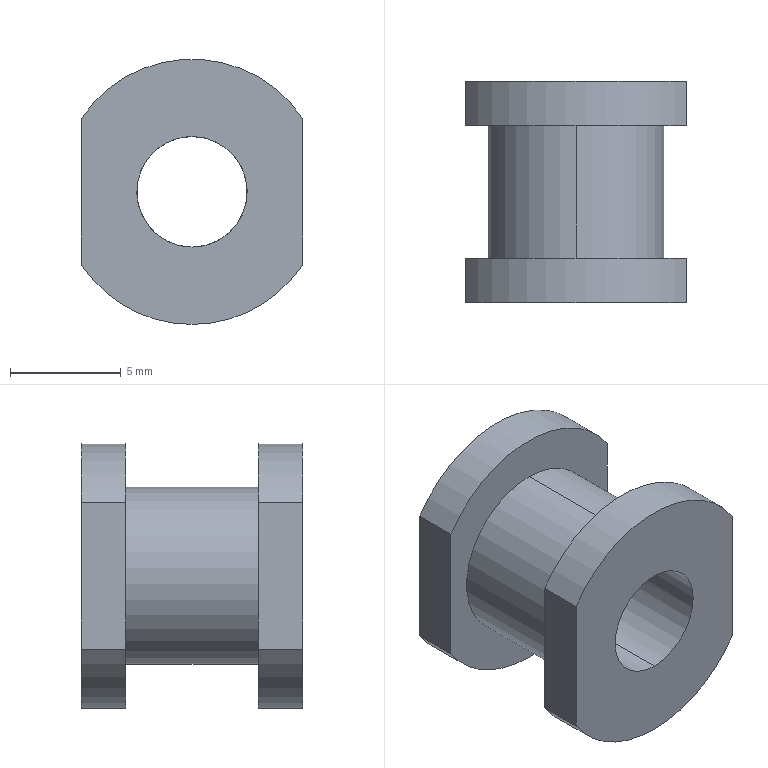Component | SolidWorks | F01AE00021-D54313-1 | 1 solid | 18 faces | box 10 x 10 x 12 mm | volume 522 mm3 | cylinder 10 | plane 8 | commonest cylinder face diameters 12 x6 5 x2 8 x2
build123d program:
from build123d import *

# Parameters (mm, degrees)
CUT_EXTRUDE1_DEPTH              = 10
M5_TAPPED_HOLE1_D               = 4.2
M5_TAPPED_HOLE1_DEPTH           = 12.4
M5_TAPPED_HOLE1_TIP             = 1.262
M5_THREADMAJORRELIEF_DEPTH      = 13.689
M5_THREADMAJORRELIEF_DEPTH_BACK = 13.689
M5_THREADMAJORRELIEF_SKETCH_R   = 2.5


with BuildPart() as part:
    # Sketch1 → Revolve1 (revolve)
    with BuildSketch(Plane.XY, mode=Mode.PRIVATE) as revolve1_sk:
        Polygon((2, 10), (2, 0), (6, 0), (6, 2), (4, 2), (4, 8), (6, 8), (6, 10), align=None)
    revolve(revolve1_sk.sketch.rotate(Axis((0, 0, 0), (0, 1, 0)), 90), axis=Axis((0, 0, 0), (0, 1, 0)))

    # Sketch2 → Cut-Extrude1 (cut)
    with BuildSketch(Plane(origin=(0, 10, 0), x_dir=(1, 0, 0), z_dir=(0, 1, 0))):
        with BuildLine():
            Line((-5, 3.317), (-5, -3.317))
            ThreePointArc((-5, -3.317), (-6, 0), (-5, 3.317))
        make_face()
        with BuildLine():
            Line((5, 3.317), (5, -3.317))
            ThreePointArc((5, -3.317), (6, 0), (5, 3.317))
        make_face()
    extrude(amount=-CUT_EXTRUDE1_DEPTH, mode=Mode.SUBTRACT)

    # M5 Tapped Hole1
    with Locations(Plane(origin=(0, 10, 0), x_dir=(1, 0, 0), z_dir=(0, 1, 0))):
        with Locations((0, 0)):
            Hole(M5_TAPPED_HOLE1_D / 2, depth=M5_TAPPED_HOLE1_DEPTH)
            with Locations((0, 0, -(M5_TAPPED_HOLE1_DEPTH + M5_TAPPED_HOLE1_TIP / 2))):  # 118° drill point
                Cone(0, M5_TAPPED_HOLE1_D / 2, M5_TAPPED_HOLE1_TIP, mode=Mode.SUBTRACT)

    # M5_ThreadMajorRelief_Sketch → M5_ThreadMajorRelief (cut, two sides: drawn at the far end of the back side and taken through both)
    with BuildSketch(Plane(origin=(0, 0, 0), x_dir=(1, 0, 0), z_dir=(0, 1, 0)).offset(-M5_THREADMAJORRELIEF_DEPTH_BACK)):
        with Locations(Location((0, 0, 0), (0, 0, 270))):
            Circle(M5_THREADMAJORRELIEF_SKETCH_R)
    extrude(amount=M5_THREADMAJORRELIEF_DEPTH + M5_THREADMAJORRELIEF_DEPTH_BACK, mode=Mode.SUBTRACT)


solid = part.part

# Placed as in the assembly
solid = solid.moved(Location((272.334, 153.205, 237.764), (0, 0, 0)))
STEP:
#1=COLOUR_RGB('',0.7922,0.8196,0.9333);
#2=FILL_AREA_STYLE_COLOUR('',#1);
#3=FILL_AREA_STYLE('',(#2));
#4=SURFACE_STYLE_FILL_AREA(#3);
#5=SURFACE_SIDE_STYLE('',(#4));
#6=SURFACE_STYLE_USAGE(.BOTH.,#5);
#7=PRESENTATION_STYLE_ASSIGNMENT((#6));
#8=CARTESIAN_POINT('',(10.722,6.032,9.262));
#9=VERTEX_POINT('',#8);
#10=CARTESIAN_POINT('',(10.722,6.032,9.459));
#11=VERTEX_POINT('',#10);
#12=CARTESIAN_POINT('',(10.722,6.032,9.262));
#13=CARTESIAN_POINT('',(10.709,6.032,9.262));
#14=CARTESIAN_POINT('',(10.696,6.032,9.265));
#15=CARTESIAN_POINT('',(10.672,6.032,9.275));
#16=CARTESIAN_POINT('',(10.661,6.032,9.282));
#17=CARTESIAN_POINT('',(10.643,6.032,9.3));
#18=CARTESIAN_POINT('',(10.636,6.032,9.311));
#19=CARTESIAN_POINT('',(10.626,6.032,9.335));
#20=CARTESIAN_POINT('',(10.623,6.032,9.348));
#21=CARTESIAN_POINT('',(10.623,6.032,9.374));
#22=CARTESIAN_POINT('',(10.626,6.032,9.386));
#23=CARTESIAN_POINT('',(10.636,6.032,9.411));
#24=CARTESIAN_POINT('',(10.643,6.032,9.421));
#25=CARTESIAN_POINT('',(10.661,6.032,9.44));
#26=CARTESIAN_POINT('',(10.672,6.032,9.447));
#27=CARTESIAN_POINT('',(10.696,6.032,9.457));
#28=CARTESIAN_POINT('',(10.709,6.032,9.459));
#29=CARTESIAN_POINT('',(10.722,6.032,9.459));
#30=B_SPLINE_CURVE_WITH_KNOTS('',3,(#12,#13,#14,#15,#16,#17,#18,#19,#20,#21,#22,#23,#24,#25,#26,#27,#28,#29),.UNSPECIFIED.,.F.,.F.,(4,2,2,2,2,2,2,2,4),(0.5,0.5625,0.625,0.6875,0.75,0.8125,0.875,0.9375,1.),.UNSPECIFIED.);
#31=EDGE_CURVE('',#9,#11,#30,.T.);
#32=ORIENTED_EDGE('',*,*,#31,.F.);
#33=CARTESIAN_POINT('',(10.722,6.425,9.262));
#34=VERTEX_POINT('',#33);
#35=CARTESIAN_POINT('',(10.722,6.032,9.262));
#36=DIRECTION('',(0.,1.,0.));
#37=VECTOR('',#36,39.37);
#38=LINE('',#35,#37);
#39=EDGE_CURVE('',#9,#34,#38,.T.);
#40=ORIENTED_EDGE('',*,*,#39,.T.);
#41=CARTESIAN_POINT('',(10.722,6.425,9.459));
#42=VERTEX_POINT('',#41);
#43=CARTESIAN_POINT('',(10.722,6.425,9.361));
#44=DIRECTION('',(0.,1.,0.));
#45=DIRECTION('',(0.,0.,1.));
#46=AXIS2_PLACEMENT_3D('',#43,#44,#45);
#47=CIRCLE('',#46,0.09843);
#48=EDGE_CURVE('',#34,#42,#47,.T.);
#49=ORIENTED_EDGE('',*,*,#48,.T.);
#50=CARTESIAN_POINT('',(10.722,6.032,9.459));
#51=DIRECTION('',(0.,1.,0.));
#52=VECTOR('',#51,39.37);
#53=LINE('',#50,#52);
#54=EDGE_CURVE('',#11,#42,#53,.T.);
#55=ORIENTED_EDGE('',*,*,#54,.F.);
#56=EDGE_LOOP('',(#32,#40,#49,#55));
#57=FACE_OUTER_BOUND('',#56,.T.);
#58=CARTESIAN_POINT('',(10.722,6.032,9.361));
#59=DIRECTION('',(0.,1.,0.));
#60=DIRECTION('',(0.,0.,1.));
#61=AXIS2_PLACEMENT_3D('',#58,#59,#60);
#62=CYLINDRICAL_SURFACE('',#61,0.09843);
#63=ADVANCED_FACE('',(#57),#62,.F.);
#64=CARTESIAN_POINT('',(10.722,6.347,9.203));
#65=VERTEX_POINT('',#64);
#66=CARTESIAN_POINT('',(10.722,6.347,9.518));
#67=VERTEX_POINT('',#66);
#68=CARTESIAN_POINT('',(10.722,6.347,9.361));
#69=DIRECTION('',(0.,-1.,0.));
#70=DIRECTION('',(0.,0.,-1.));
#71=AXIS2_PLACEMENT_3D('',#68,#69,#70);
#72=CIRCLE('',#71,0.1575);
#73=EDGE_CURVE('',#65,#67,#72,.T.);
#74=ORIENTED_EDGE('',*,*,#73,.T.);
#75=CARTESIAN_POINT('',(10.722,6.11,9.518));
#76=VERTEX_POINT('',#75);
#77=CARTESIAN_POINT('',(10.722,6.032,9.518));
#78=DIRECTION('',(0.,-1.,0.));
#79=VECTOR('',#78,39.37);
#80=LINE('',#77,#79);
#81=EDGE_CURVE('',#67,#76,#80,.T.);
#82=ORIENTED_EDGE('',*,*,#81,.T.);
#83=CARTESIAN_POINT('',(10.722,6.11,9.203));
#84=VERTEX_POINT('',#83);
#85=CARTESIAN_POINT('',(10.722,6.11,9.361));
#86=DIRECTION('',(0.,-1.,0.));
#87=DIRECTION('',(0.,0.,-1.));
#88=AXIS2_PLACEMENT_3D('',#85,#86,#87);
#89=CIRCLE('',#88,0.1575);
#90=EDGE_CURVE('',#84,#76,#89,.T.);
#91=ORIENTED_EDGE('',*,*,#90,.F.);
#92=CARTESIAN_POINT('',(10.722,6.032,9.203));
#93=DIRECTION('',(0.,-1.,0.));
#94=VECTOR('',#93,39.37);
#95=LINE('',#92,#94);
#96=EDGE_CURVE('',#65,#84,#95,.T.);
#97=ORIENTED_EDGE('',*,*,#96,.F.);
#98=EDGE_LOOP('',(#74,#82,#91,#97));
#99=FACE_OUTER_BOUND('',#98,.T.);
#100=CARTESIAN_POINT('',(10.722,6.032,9.361));
#101=DIRECTION('',(0.,-1.,0.));
#102=DIRECTION('',(0.,0.,-1.));
#103=AXIS2_PLACEMENT_3D('',#100,#101,#102);
#104=CYLINDRICAL_SURFACE('',#103,0.1575);
#105=ADVANCED_FACE('',(#99),#104,.T.);
#106=CARTESIAN_POINT('',(10.525,6.425,9.23));
#107=VERTEX_POINT('',#106);
#108=CARTESIAN_POINT('',(10.722,6.425,9.125));
#109=VERTEX_POINT('',#108);
#110=CARTESIAN_POINT('',(10.722,6.425,9.361));
#111=DIRECTION('',(0.,-1.,0.));
#112=DIRECTION('',(0.,0.,-1.));
#113=AXIS2_PLACEMENT_3D('',#110,#111,#112);
#114=CIRCLE('',#113,0.2362);
#115=EDGE_CURVE('',#107,#109,#114,.T.);
#116=ORIENTED_EDGE('',*,*,#115,.T.);
#117=CARTESIAN_POINT('',(10.722,6.347,9.125));
#118=VERTEX_POINT('',#117);
#119=CARTESIAN_POINT('',(10.722,6.032,9.125));
#120=DIRECTION('',(0.,-1.,0.));
#121=VECTOR('',#120,39.37);
#122=LINE('',#119,#121);
#123=EDGE_CURVE('',#109,#118,#122,.T.);
#124=ORIENTED_EDGE('',*,*,#123,.T.);
#125=CARTESIAN_POINT('',(10.525,6.347,9.23));
#126=VERTEX_POINT('',#125);
#127=CARTESIAN_POINT('',(10.722,6.347,9.361));
#128=DIRECTION('',(0.,-1.,0.));
#129=DIRECTION('',(0.,0.,-1.));
#130=AXIS2_PLACEMENT_3D('',#127,#128,#129);
#131=CIRCLE('',#130,0.2362);
#132=EDGE_CURVE('',#126,#118,#131,.T.);
#133=ORIENTED_EDGE('',*,*,#132,.F.);
#134=CARTESIAN_POINT('',(10.525,6.032,9.23));
#135=DIRECTION('',(0.,-1.,0.));
#136=VECTOR('',#135,39.37);
#137=LINE('',#134,#136);
#138=EDGE_CURVE('',#107,#126,#137,.T.);
#139=ORIENTED_EDGE('',*,*,#138,.F.);
#140=EDGE_LOOP('',(#116,#124,#133,#139));
#141=FACE_OUTER_BOUND('',#140,.T.);
#142=CARTESIAN_POINT('',(10.722,6.032,9.361));
#143=DIRECTION('',(0.,-1.,0.));
#144=DIRECTION('',(0.,0.,-1.));
#145=AXIS2_PLACEMENT_3D('',#142,#143,#144);
#146=CYLINDRICAL_SURFACE('',#145,0.2362);
#147=ADVANCED_FACE('',(#141),#146,.T.);
#148=CARTESIAN_POINT('',(10.525,6.11,9.23));
#149=VERTEX_POINT('',#148);
#150=CARTESIAN_POINT('',(10.722,6.11,9.125));
#151=VERTEX_POINT('',#150);
#152=CARTESIAN_POINT('',(10.722,6.11,9.361));
#153=DIRECTION('',(0.,-1.,0.));
#154=DIRECTION('',(0.,0.,-1.));
#155=AXIS2_PLACEMENT_3D('',#152,#153,#154);
#156=CIRCLE('',#155,0.2362);
#157=EDGE_CURVE('',#149,#151,#156,.T.);
#158=ORIENTED_EDGE('',*,*,#157,.T.);
#159=CARTESIAN_POINT('',(10.722,6.032,9.125));
#160=VERTEX_POINT('',#159);
#161=CARTESIAN_POINT('',(10.722,6.032,9.125));
#162=DIRECTION('',(0.,-1.,0.));
#163=VECTOR('',#162,39.37);
#164=LINE('',#161,#163);
#165=EDGE_CURVE('',#151,#160,#164,.T.);
#166=ORIENTED_EDGE('',*,*,#165,.T.);
#167=CARTESIAN_POINT('',(10.525,6.032,9.23));
#168=VERTEX_POINT('',#167);
#169=CARTESIAN_POINT('',(10.722,6.032,9.361));
#170=DIRECTION('',(0.,-1.,0.));
#171=DIRECTION('',(0.,0.,-1.));
#172=AXIS2_PLACEMENT_3D('',#169,#170,#171);
#173=CIRCLE('',#172,0.2362);
#174=EDGE_CURVE('',#168,#160,#173,.T.);
#175=ORIENTED_EDGE('',*,*,#174,.F.);
#176=CARTESIAN_POINT('',(10.525,6.032,9.23));
#177=DIRECTION('',(0.,1.,0.));
#178=VECTOR('',#177,39.37);
#179=LINE('',#176,#178);
#180=EDGE_CURVE('',#168,#149,#179,.T.);
#181=ORIENTED_EDGE('',*,*,#180,.T.);
#182=EDGE_LOOP('',(#158,#166,#175,#181));
#183=FACE_OUTER_BOUND('',#182,.T.);
#184=CARTESIAN_POINT('',(10.722,6.032,9.361));
#185=DIRECTION('',(0.,-1.,0.));
#186=DIRECTION('',(0.,0.,-1.));
#187=AXIS2_PLACEMENT_3D('',#184,#185,#186);
#188=CYLINDRICAL_SURFACE('',#187,0.2362);
#189=ADVANCED_FACE('',(#183),#188,.T.);
#190=CARTESIAN_POINT('',(10.919,6.032,9.23));
#191=VERTEX_POINT('',#190);
#192=CARTESIAN_POINT('',(10.919,6.032,9.491));
#193=VERTEX_POINT('',#192);
#194=CARTESIAN_POINT('',(10.919,6.032,9.23));
#195=DIRECTION('',(0.,0.,1.));
#196=VECTOR('',#195,39.37);
#197=LINE('',#194,#196);
#198=EDGE_CURVE('',#191,#193,#197,.T.);
#199=ORIENTED_EDGE('',*,*,#198,.T.);
#200=CARTESIAN_POINT('',(10.525,6.032,9.491));
#201=VERTEX_POINT('',#200);
#202=CARTESIAN_POINT('',(10.722,6.032,9.361));
#203=DIRECTION('',(0.,-1.,0.));
#204=DIRECTION('',(0.,0.,-1.));
#205=AXIS2_PLACEMENT_3D('',#202,#203,#204);
#206=CIRCLE('',#205,0.2362);
#207=EDGE_CURVE('',#193,#201,#206,.T.);
#208=ORIENTED_EDGE('',*,*,#207,.T.);
#209=CARTESIAN_POINT('',(10.525,6.032,9.23));
#210=DIRECTION('',(0.,0.,-1.));
#211=VECTOR('',#210,39.37);
#212=LINE('',#209,#211);
#213=EDGE_CURVE('',#201,#168,#212,.T.);
#214=ORIENTED_EDGE('',*,*,#213,.T.);
#215=ORIENTED_EDGE('',*,*,#174,.T.);
#216=CARTESIAN_POINT('',(10.722,6.032,9.361));
#217=DIRECTION('',(0.,-1.,0.));
#218=DIRECTION('',(0.,0.,-1.));
#219=AXIS2_PLACEMENT_3D('',#216,#217,#218);
#220=CIRCLE('',#219,0.2362);
#221=EDGE_CURVE('',#160,#191,#220,.T.);
#222=ORIENTED_EDGE('',*,*,#221,.T.);
#223=EDGE_LOOP('',(#199,#208,#214,#215,#222));
#224=FACE_OUTER_BOUND('',#223,.T.);
#225=CARTESIAN_POINT('',(10.722,6.032,9.459));
#226=CARTESIAN_POINT('',(10.735,6.032,9.459));
#227=CARTESIAN_POINT('',(10.747,6.032,9.457));
#228=CARTESIAN_POINT('',(10.772,6.032,9.447));
#229=CARTESIAN_POINT('',(10.782,6.032,9.44));
#230=CARTESIAN_POINT('',(10.801,6.032,9.421));
#231=CARTESIAN_POINT('',(10.808,6.032,9.411));
#232=CARTESIAN_POINT('',(10.818,6.032,9.386));
#233=CARTESIAN_POINT('',(10.82,6.032,9.374));
#234=CARTESIAN_POINT('',(10.82,6.032,9.348));
#235=CARTESIAN_POINT('',(10.818,6.032,9.335));
#236=CARTESIAN_POINT('',(10.808,6.032,9.311));
#237=CARTESIAN_POINT('',(10.801,6.032,9.3));
#238=CARTESIAN_POINT('',(10.782,6.032,9.282));
#239=CARTESIAN_POINT('',(10.772,6.032,9.275));
#240=CARTESIAN_POINT('',(10.747,6.032,9.265));
#241=CARTESIAN_POINT('',(10.735,6.032,9.262));
#242=CARTESIAN_POINT('',(10.722,6.032,9.262));
#243=B_SPLINE_CURVE_WITH_KNOTS('',3,(#225,#226,#227,#228,#229,#230,#231,#232,#233,#234,#235,#236,#237,#238,#239,#240,#241,#242),.UNSPECIFIED.,.F.,.F.,(4,2,2,2,2,2,2,2,4),(0.,0.0625,0.125,0.1875,0.25,0.3125,0.375,0.4375,0.5),.UNSPECIFIED.);
#244=EDGE_CURVE('',#11,#9,#243,.T.);
#245=ORIENTED_EDGE('',*,*,#244,.T.);
#246=ORIENTED_EDGE('',*,*,#31,.T.);
#247=EDGE_LOOP('',(#245,#246));
#248=FACE_BOUND('',#247,.T.);
#249=CARTESIAN_POINT('',(10.801,6.032,9.361));
#250=DIRECTION('',(0.,-1.,0.));
#251=DIRECTION('',(0.,0.,-1.));
#252=AXIS2_PLACEMENT_3D('',#249,#250,#251);
#253=PLANE('',#252);
#254=ADVANCED_FACE('',(#224,#248),#253,.T.);
#255=ORIENTED_EDGE('',*,*,#165,.F.);
#256=CARTESIAN_POINT('',(10.919,6.11,9.23));
#257=VERTEX_POINT('',#256);
#258=CARTESIAN_POINT('',(10.722,6.11,9.361));
#259=DIRECTION('',(0.,-1.,0.));
#260=DIRECTION('',(0.,0.,-1.));
#261=AXIS2_PLACEMENT_3D('',#258,#259,#260);
#262=CIRCLE('',#261,0.2362);
#263=EDGE_CURVE('',#151,#257,#262,.T.);
#264=ORIENTED_EDGE('',*,*,#263,.T.);
#265=CARTESIAN_POINT('',(10.919,6.032,9.23));
#266=DIRECTION('',(0.,1.,0.));
#267=VECTOR('',#266,39.37);
#268=LINE('',#265,#267);
#269=EDGE_CURVE('',#191,#257,#268,.T.);
#270=ORIENTED_EDGE('',*,*,#269,.F.);
#271=ORIENTED_EDGE('',*,*,#221,.F.);
#272=EDGE_LOOP('',(#255,#264,#270,#271));
#273=FACE_OUTER_BOUND('',#272,.T.);
#274=CARTESIAN_POINT('',(10.722,6.032,9.361));
#275=DIRECTION('',(0.,-1.,0.));
#276=DIRECTION('',(0.,0.,-1.));
#277=AXIS2_PLACEMENT_3D('',#274,#275,#276);
#278=CYLINDRICAL_SURFACE('',#277,0.2362);
#279=ADVANCED_FACE('',(#273),#278,.T.);
#280=ORIENTED_EDGE('',*,*,#123,.F.);
#281=CARTESIAN_POINT('',(10.919,6.425,9.23));
#282=VERTEX_POINT('',#281);
#283=CARTESIAN_POINT('',(10.722,6.425,9.361));
#284=DIRECTION('',(0.,-1.,0.));
#285=DIRECTION('',(0.,0.,-1.));
#286=AXIS2_PLACEMENT_3D('',#283,#284,#285);
#287=CIRCLE('',#286,0.2362);
#288=EDGE_CURVE('',#109,#282,#287,.T.);
#289=ORIENTED_EDGE('',*,*,#288,.T.);
#290=CARTESIAN_POINT('',(10.919,6.347,9.23));
#291=VERTEX_POINT('',#290);
#292=CARTESIAN_POINT('',(10.919,6.032,9.23));
#293=DIRECTION('',(0.,1.,0.));
#294=VECTOR('',#293,39.37);
#295=LINE('',#292,#294);
#296=EDGE_CURVE('',#291,#282,#295,.T.);
#297=ORIENTED_EDGE('',*,*,#296,.F.);
#298=CARTESIAN_POINT('',(10.722,6.347,9.361));
#299=DIRECTION('',(0.,-1.,0.));
#300=DIRECTION('',(0.,0.,-1.));
#301=AXIS2_PLACEMENT_3D('',#298,#299,#300);
#302=CIRCLE('',#301,0.2362);
#303=EDGE_CURVE('',#118,#291,#302,.T.);
#304=ORIENTED_EDGE('',*,*,#303,.F.);
#305=EDGE_LOOP('',(#280,#289,#297,#304));
#306=FACE_OUTER_BOUND('',#305,.T.);
#307=CARTESIAN_POINT('',(10.722,6.032,9.361));
#308=DIRECTION('',(0.,-1.,0.));
#309=DIRECTION('',(0.,0.,-1.));
#310=AXIS2_PLACEMENT_3D('',#307,#308,#309);
#311=CYLINDRICAL_SURFACE('',#310,0.2362);
#312=ADVANCED_FACE('',(#306),#311,.T.);
#313=CARTESIAN_POINT('',(10.722,6.425,9.361));
#314=DIRECTION('',(0.,1.,0.));
#315=DIRECTION('',(0.,0.,1.));
#316=AXIS2_PLACEMENT_3D('',#313,#314,#315);
#317=CIRCLE('',#316,0.09843);
#318=EDGE_CURVE('',#42,#34,#317,.T.);
#319=ORIENTED_EDGE('',*,*,#318,.F.);
#320=ORIENTED_EDGE('',*,*,#48,.F.);
#321=EDGE_LOOP('',(#319,#320));
#322=FACE_BOUND('',#321,.T.);
#323=CARTESIAN_POINT('',(10.919,6.425,9.491));
#324=VERTEX_POINT('',#323);
#325=CARTESIAN_POINT('',(10.919,6.425,9.23));
#326=DIRECTION('',(0.,0.,1.));
#327=VECTOR('',#326,39.37);
#328=LINE('',#325,#327);
#329=EDGE_CURVE('',#282,#324,#328,.T.);
#330=ORIENTED_EDGE('',*,*,#329,.F.);
#331=ORIENTED_EDGE('',*,*,#288,.F.);
#332=ORIENTED_EDGE('',*,*,#115,.F.);
#333=CARTESIAN_POINT('',(10.525,6.425,9.491));
#334=VERTEX_POINT('',#333);
#335=CARTESIAN_POINT('',(10.525,6.425,9.23));
#336=DIRECTION('',(0.,0.,-1.));
#337=VECTOR('',#336,39.37);
#338=LINE('',#335,#337);
#339=EDGE_CURVE('',#334,#107,#338,.T.);
#340=ORIENTED_EDGE('',*,*,#339,.F.);
#341=CARTESIAN_POINT('',(10.722,6.425,9.361));
#342=DIRECTION('',(0.,-1.,0.));
#343=DIRECTION('',(0.,0.,-1.));
#344=AXIS2_PLACEMENT_3D('',#341,#342,#343);
#345=CIRCLE('',#344,0.2362);
#346=EDGE_CURVE('',#324,#334,#345,.T.);
#347=ORIENTED_EDGE('',*,*,#346,.F.);
#348=EDGE_LOOP('',(#330,#331,#332,#340,#347));
#349=FACE_OUTER_BOUND('',#348,.T.);
#350=CARTESIAN_POINT('',(10.958,6.425,9.361));
#351=DIRECTION('',(0.,1.,0.));
#352=DIRECTION('',(0.,0.,1.));
#353=AXIS2_PLACEMENT_3D('',#350,#351,#352);
#354=PLANE('',#353);
#355=ADVANCED_FACE('',(#322,#349),#354,.T.);
#356=CARTESIAN_POINT('',(10.919,6.11,9.491));
#357=VERTEX_POINT('',#356);
#358=CARTESIAN_POINT('',(10.919,6.032,9.491));
#359=DIRECTION('',(0.,1.,0.));
#360=VECTOR('',#359,39.37);
#361=LINE('',#358,#360);
#362=EDGE_CURVE('',#193,#357,#361,.T.);
#363=ORIENTED_EDGE('',*,*,#362,.T.);
#364=CARTESIAN_POINT('',(10.525,6.11,9.491));
#365=VERTEX_POINT('',#364);
#366=CARTESIAN_POINT('',(10.722,6.11,9.361));
#367=DIRECTION('',(0.,-1.,0.));
#368=DIRECTION('',(0.,0.,-1.));
#369=AXIS2_PLACEMENT_3D('',#366,#367,#368);
#370=CIRCLE('',#369,0.2362);
#371=EDGE_CURVE('',#357,#365,#370,.T.);
#372=ORIENTED_EDGE('',*,*,#371,.T.);
#373=CARTESIAN_POINT('',(10.525,6.032,9.491));
#374=DIRECTION('',(0.,1.,0.));
#375=VECTOR('',#374,39.37);
#376=LINE('',#373,#375);
#377=EDGE_CURVE('',#201,#365,#376,.T.);
#378=ORIENTED_EDGE('',*,*,#377,.F.);
#379=ORIENTED_EDGE('',*,*,#207,.F.);
#380=EDGE_LOOP('',(#363,#372,#378,#379));
#381=FACE_OUTER_BOUND('',#380,.T.);
#382=CARTESIAN_POINT('',(10.722,6.032,9.361));
#383=DIRECTION('',(0.,-1.,0.));
#384=DIRECTION('',(0.,0.,-1.));
#385=AXIS2_PLACEMENT_3D('',#382,#383,#384);
#386=CYLINDRICAL_SURFACE('',#385,0.2362);
#387=ADVANCED_FACE('',(#381),#386,.T.);
#388=CARTESIAN_POINT('',(10.919,6.11,9.361));
#389=DIRECTION('',(0.,0.,1.));
#390=VECTOR('',#389,39.37);
#391=LINE('',#388,#390);
#392=EDGE_CURVE('',#257,#357,#391,.T.);
#393=ORIENTED_EDGE('',*,*,#392,.F.);
#394=ORIENTED_EDGE('',*,*,#263,.F.);
#395=ORIENTED_EDGE('',*,*,#157,.F.);
#396=CARTESIAN_POINT('',(10.525,6.11,9.361));
#397=DIRECTION('',(0.,0.,-1.));
#398=VECTOR('',#397,39.37);
#399=LINE('',#396,#398);
#400=EDGE_CURVE('',#365,#149,#399,.T.);
#401=ORIENTED_EDGE('',*,*,#400,.F.);
#402=ORIENTED_EDGE('',*,*,#371,.F.);
#403=EDGE_LOOP('',(#393,#394,#395,#401,#402));
#404=FACE_OUTER_BOUND('',#403,.T.);
#405=ORIENTED_EDGE('',*,*,#90,.T.);
#406=CARTESIAN_POINT('',(10.722,6.11,9.361));
#407=DIRECTION('',(0.,-1.,0.));
#408=DIRECTION('',(0.,0.,-1.));
#409=AXIS2_PLACEMENT_3D('',#406,#407,#408);
#410=CIRCLE('',#409,0.1575);
#411=EDGE_CURVE('',#76,#84,#410,.T.);
#412=ORIENTED_EDGE('',*,*,#411,.T.);
#413=EDGE_LOOP('',(#405,#412));
#414=FACE_BOUND('',#413,.T.);
#415=CARTESIAN_POINT('',(10.958,6.11,9.361));
#416=DIRECTION('',(0.,1.,0.));
#417=DIRECTION('',(0.,0.,1.));
#418=AXIS2_PLACEMENT_3D('',#415,#416,#417);
#419=PLANE('',#418);
#420=ADVANCED_FACE('',(#404,#414),#419,.T.);
#421=ORIENTED_EDGE('',*,*,#81,.F.);
#422=CARTESIAN_POINT('',(10.722,6.347,9.361));
#423=DIRECTION('',(0.,-1.,0.));
#424=DIRECTION('',(0.,0.,-1.));
#425=AXIS2_PLACEMENT_3D('',#422,#423,#424);
#426=CIRCLE('',#425,0.1575);
#427=EDGE_CURVE('',#67,#65,#426,.T.);
#428=ORIENTED_EDGE('',*,*,#427,.T.);
#429=ORIENTED_EDGE('',*,*,#96,.T.);
#430=ORIENTED_EDGE('',*,*,#411,.F.);
#431=EDGE_LOOP('',(#421,#428,#429,#430));
#432=FACE_OUTER_BOUND('',#431,.T.);
#433=CARTESIAN_POINT('',(10.722,6.032,9.361));
#434=DIRECTION('',(0.,-1.,0.));
#435=DIRECTION('',(0.,0.,-1.));
#436=AXIS2_PLACEMENT_3D('',#433,#434,#435);
#437=CYLINDRICAL_SURFACE('',#436,0.1575);
#438=ADVANCED_FACE('',(#432),#437,.T.);
#439=CARTESIAN_POINT('',(10.919,6.347,9.491));
#440=VERTEX_POINT('',#439);
#441=CARTESIAN_POINT('',(10.919,6.347,9.361));
#442=DIRECTION('',(0.,0.,-1.));
#443=VECTOR('',#442,39.37);
#444=LINE('',#441,#443);
#445=EDGE_CURVE('',#440,#291,#444,.T.);
#446=ORIENTED_EDGE('',*,*,#445,.F.);
#447=CARTESIAN_POINT('',(10.525,6.347,9.491));
#448=VERTEX_POINT('',#447);
#449=CARTESIAN_POINT('',(10.722,6.347,9.361));
#450=DIRECTION('',(0.,-1.,0.));
#451=DIRECTION('',(0.,0.,-1.));
#452=AXIS2_PLACEMENT_3D('',#449,#450,#451);
#453=CIRCLE('',#452,0.2362);
#454=EDGE_CURVE('',#440,#448,#453,.T.);
#455=ORIENTED_EDGE('',*,*,#454,.T.);
#456=CARTESIAN_POINT('',(10.525,6.347,9.361));
#457=DIRECTION('',(0.,0.,1.));
#458=VECTOR('',#457,39.37);
#459=LINE('',#456,#458);
#460=EDGE_CURVE('',#126,#448,#459,.T.);
#461=ORIENTED_EDGE('',*,*,#460,.F.);
#462=ORIENTED_EDGE('',*,*,#132,.T.);
#463=ORIENTED_EDGE('',*,*,#303,.T.);
#464=EDGE_LOOP('',(#446,#455,#461,#462,#463));
#465=FACE_OUTER_BOUND('',#464,.T.);
#466=ORIENTED_EDGE('',*,*,#73,.F.);
#467=ORIENTED_EDGE('',*,*,#427,.F.);
#468=EDGE_LOOP('',(#466,#467));
#469=FACE_BOUND('',#468,.T.);
#470=CARTESIAN_POINT('',(10.879,6.347,9.361));
#471=DIRECTION('',(0.,-1.,0.));
#472=DIRECTION('',(0.,0.,-1.));
#473=AXIS2_PLACEMENT_3D('',#470,#471,#472);
#474=PLANE('',#473);
#475=ADVANCED_FACE('',(#465,#469),#474,.T.);
#476=CARTESIAN_POINT('',(10.919,6.032,9.491));
#477=DIRECTION('',(0.,-1.,0.));
#478=VECTOR('',#477,39.37);
#479=LINE('',#476,#478);
#480=EDGE_CURVE('',#324,#440,#479,.T.);
#481=ORIENTED_EDGE('',*,*,#480,.F.);
#482=ORIENTED_EDGE('',*,*,#346,.T.);
#483=CARTESIAN_POINT('',(10.525,6.032,9.491));
#484=DIRECTION('',(0.,1.,0.));
#485=VECTOR('',#484,39.37);
#486=LINE('',#483,#485);
#487=EDGE_CURVE('',#448,#334,#486,.T.);
#488=ORIENTED_EDGE('',*,*,#487,.F.);
#489=ORIENTED_EDGE('',*,*,#454,.F.);
#490=EDGE_LOOP('',(#481,#482,#488,#489));
#491=FACE_OUTER_BOUND('',#490,.T.);
#492=CARTESIAN_POINT('',(10.722,6.032,9.361));
#493=DIRECTION('',(0.,-1.,0.));
#494=DIRECTION('',(0.,0.,-1.));
#495=AXIS2_PLACEMENT_3D('',#492,#493,#494);
#496=CYLINDRICAL_SURFACE('',#495,0.2362);
#497=ADVANCED_FACE('',(#491),#496,.T.);
#498=ORIENTED_EDGE('',*,*,#460,.T.);
#499=ORIENTED_EDGE('',*,*,#487,.T.);
#500=ORIENTED_EDGE('',*,*,#339,.T.);
#501=ORIENTED_EDGE('',*,*,#138,.T.);
#502=EDGE_LOOP('',(#498,#499,#500,#501));
#503=FACE_OUTER_BOUND('',#502,.T.);
#504=CARTESIAN_POINT('',(10.525,6.032,9.23));
#505=DIRECTION('',(1.,0.,0.));
#506=DIRECTION('',(0.,0.,-1.));
#507=AXIS2_PLACEMENT_3D('',#504,#505,#506);
#508=PLANE('',#507);
#509=ADVANCED_FACE('',(#503),#508,.F.);
#510=ORIENTED_EDGE('',*,*,#400,.T.);
#511=ORIENTED_EDGE('',*,*,#180,.F.);
#512=ORIENTED_EDGE('',*,*,#213,.F.);
#513=ORIENTED_EDGE('',*,*,#377,.T.);
#514=EDGE_LOOP('',(#510,#511,#512,#513));
#515=FACE_OUTER_BOUND('',#514,.T.);
#516=CARTESIAN_POINT('',(10.525,6.032,9.23));
#517=DIRECTION('',(1.,0.,0.));
#518=DIRECTION('',(0.,0.,-1.));
#519=AXIS2_PLACEMENT_3D('',#516,#517,#518);
#520=PLANE('',#519);
#521=ADVANCED_FACE('',(#515),#520,.F.);
#522=ORIENTED_EDGE('',*,*,#445,.T.);
#523=ORIENTED_EDGE('',*,*,#296,.T.);
#524=ORIENTED_EDGE('',*,*,#329,.T.);
#525=ORIENTED_EDGE('',*,*,#480,.T.);
#526=EDGE_LOOP('',(#522,#523,#524,#525));
#527=FACE_OUTER_BOUND('',#526,.T.);
#528=CARTESIAN_POINT('',(10.919,6.032,9.23));
#529=DIRECTION('',(-1.,0.,0.));
#530=DIRECTION('',(0.,0.,1.));
#531=AXIS2_PLACEMENT_3D('',#528,#529,#530);
#532=PLANE('',#531);
#533=ADVANCED_FACE('',(#527),#532,.F.);
#534=ORIENTED_EDGE('',*,*,#392,.T.);
#535=ORIENTED_EDGE('',*,*,#362,.F.);
#536=ORIENTED_EDGE('',*,*,#198,.F.);
#537=ORIENTED_EDGE('',*,*,#269,.T.);
#538=EDGE_LOOP('',(#534,#535,#536,#537));
#539=FACE_OUTER_BOUND('',#538,.T.);
#540=CARTESIAN_POINT('',(10.919,6.032,9.23));
#541=DIRECTION('',(-1.,0.,0.));
#542=DIRECTION('',(0.,0.,1.));
#543=AXIS2_PLACEMENT_3D('',#540,#541,#542);
#544=PLANE('',#543);
#545=ADVANCED_FACE('',(#539),#544,.F.);
#546=ORIENTED_EDGE('',*,*,#39,.F.);
#547=ORIENTED_EDGE('',*,*,#244,.F.);
#548=ORIENTED_EDGE('',*,*,#54,.T.);
#549=ORIENTED_EDGE('',*,*,#318,.T.);
#550=EDGE_LOOP('',(#546,#547,#548,#549));
#551=FACE_OUTER_BOUND('',#550,.T.);
#552=CARTESIAN_POINT('',(10.722,6.032,9.361));
#553=DIRECTION('',(0.,1.,0.));
#554=DIRECTION('',(0.,0.,1.));
#555=AXIS2_PLACEMENT_3D('',#552,#553,#554);
#556=CYLINDRICAL_SURFACE('',#555,0.09843);
#557=ADVANCED_FACE('',(#551),#556,.F.);
#558=CLOSED_SHELL('',(#63,#105,#147,#189,#254,#279,#312,#355,#387,#420,#438,#475,#497,#509,#521,#533,#545,#557));
#559=MANIFOLD_SOLID_BREP('',#558);
#560=STYLED_ITEM('',(#7),#559);
#561=PRESENTATION_LAYER_ASSIGNMENT('','',(#560));
#562=(LENGTH_UNIT()NAMED_UNIT(*)SI_UNIT($,.METRE.));
#563=LENGTH_MEASURE_WITH_UNIT(LENGTH_MEASURE(0.0254),#562);
#564=DIMENSIONAL_EXPONENTS(1.,0.,0.,0.,0.,0.,0.);
#565=(CONVERSION_BASED_UNIT('',#563)LENGTH_UNIT()NAMED_UNIT(#564));
#566=UNCERTAINTY_MEASURE_WITH_UNIT(LENGTH_MEASURE(0.00001),#565,'','');
#567=(NAMED_UNIT(*)PLANE_ANGLE_UNIT()SI_UNIT($,.RADIAN.));
#568=(NAMED_UNIT(*)SI_UNIT($,.STERADIAN.)SOLID_ANGLE_UNIT());
#569=(GEOMETRIC_REPRESENTATION_CONTEXT(3)GLOBAL_UNCERTAINTY_ASSIGNED_CONTEXT((#566))GLOBAL_UNIT_ASSIGNED_CONTEXT((#565,#567,#568))REPRESENTATION_CONTEXT('',''));
#570=MECHANICAL_DESIGN_GEOMETRIC_PRESENTATION_REPRESENTATION('',(#560),#569);
#571=CARTESIAN_POINT('',(0.,0.,0.));
#572=DIRECTION('',(0.,0.,1.));
#573=DIRECTION('',(1.,0.,0.));
#574=AXIS2_PLACEMENT_3D('',#571,#572,#573);
#575=(LENGTH_UNIT()NAMED_UNIT(*)SI_UNIT($,.METRE.));
#576=LENGTH_MEASURE_WITH_UNIT(LENGTH_MEASURE(0.0254),#575);
#577=DIMENSIONAL_EXPONENTS(1.,0.,0.,0.,0.,0.,0.);
#578=(CONVERSION_BASED_UNIT('',#576)LENGTH_UNIT()NAMED_UNIT(#577));
#579=UNCERTAINTY_MEASURE_WITH_UNIT(LENGTH_MEASURE(0.00001),#578,'','');
#580=(NAMED_UNIT(*)PLANE_ANGLE_UNIT()SI_UNIT($,.RADIAN.));
#581=(NAMED_UNIT(*)SI_UNIT($,.STERADIAN.)SOLID_ANGLE_UNIT());
#582=(GEOMETRIC_REPRESENTATION_CONTEXT(3)GLOBAL_UNCERTAINTY_ASSIGNED_CONTEXT((#579))GLOBAL_UNIT_ASSIGNED_CONTEXT((#578,#580,#581))REPRESENTATION_CONTEXT('',''));
#583=ADVANCED_BREP_SHAPE_REPRESENTATION('',(#559,#574),#582);